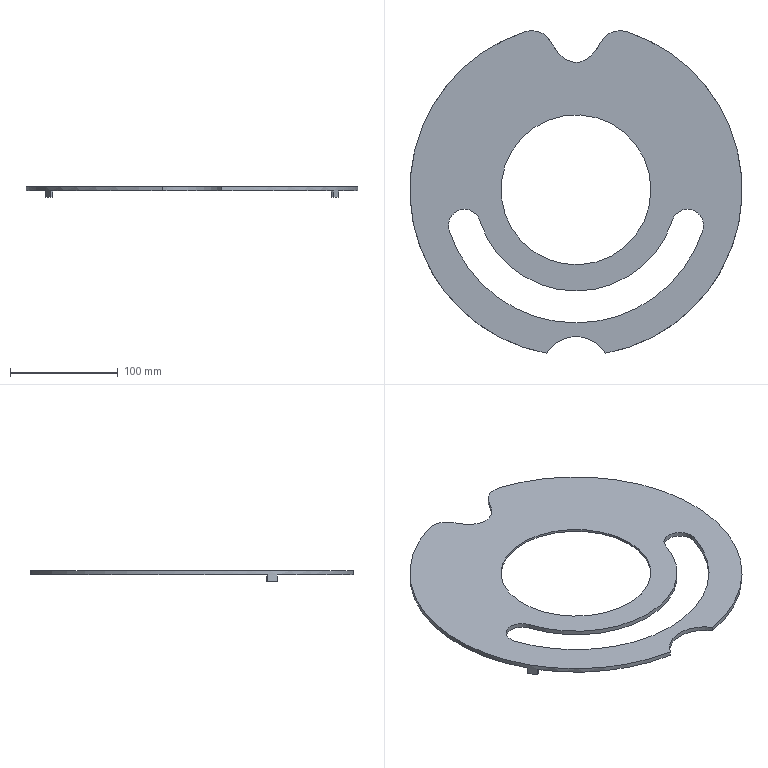Component | NX | TOP_COVER | 1 solid | 32 faces | volume 103303 mm3 | cylinder 15 | plane 11 | spline 3 | other 3 | commonest cylinder face diameters 33.617 x2 29.617 x2 304 x2 308 x2 187.556 x1 250.79 x1 246.79 x1 183.556 x1